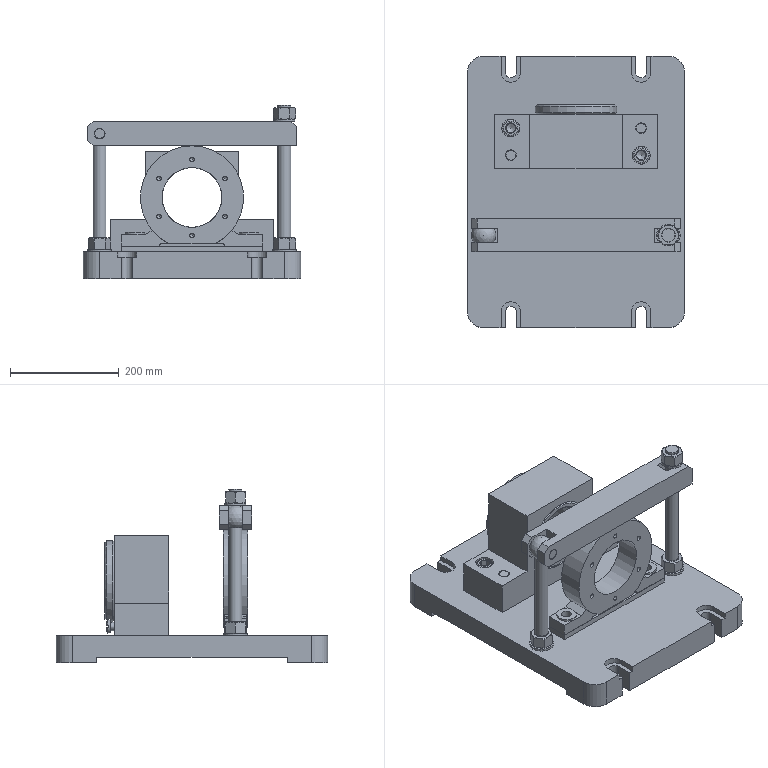Assembly | NX | mm | 21 component files | 21 solids | 393 faces | box 400 x 500 x 320 mm | volume 13709940 mm3 | plane 197 | cylinder 96 | cone 95 | torus 4 | sphere 1 | commonest cylinder face diameters 20 x16 8.5 x12 18 x9 24 x8 21.564 x6 36 x6 10 x4 16 x4
Bill of materials:
unnamed part 1 | 1 |  | Block-style support with a large horizontal cylindrical through-bore in a raised rectangular upright, sitting on a wider rectangular base with flanges extending to both sides.
GB-T848-2002,M24 | 1 |  | Flat annular ring (washer-like disc): a thin cylindrical plate with a single concentric circular through-hole and plain flat faces.
GB-T70.1-2000,M20x70 | 2 |  | Hexagon Socket Head Cap Screw, GB-T 70.1-2000,M20x70
GB-T6170_F-2000,M24x3 | 3 |  | Hexagonal prism with a central round through-hole and chamfered or curved corner faces at both ends; it looks like a hex nut.
GB-T97_1-2002,M24 | 2 |  | Flat annular ring (washer-like disc): a thin cylindrical plate with a single concentric circular through-hole and plain flat faces. Its bore is proportionally smaller than unnamed part's.
unnamed part 2 | 1 |  | Stepped cylindrical pin with a flat round head that has a straight slot, a larger-diameter shoulder below the head, a narrow neck or groove, and a smaller shank with a chamfered end.
unnamed part 3 | 1 |  | Long slender cylindrical rod ending in a rounded, roughly spherical eye with a cross-hole. Near the other end the shaft has a short reduced-diameter section, shown as one or more grooves or steps.
GB-T119.1-2000,20x60 | 1 |  | Parallel Pin, GB-T 119.1-2000,20x60
GB-T119.1-2000,20x90 | 2 |  | Parallel Pin, GB-T 119.1-2000,20x90
unnamed part 4 | 1 |  | Long flat rectangular bar with a slotted fork (clevis-style) at each end. Each fork has a transverse cross-hole, and the end corners are chamfered.
unnamed part 5 | 1 |  | Solid stepped cylindrical pin with a wider central flange or collar, cylindrical sections on both sides, small necks or undercuts next to the collar, and chamfered ends.
unnamed part 6 | 1 |  | Long slender cylindrical pin with chamfered ends and reduced-diameter sections, such as grooves or steps, near both ends.
unnamed part 7 | 1 |  | Stepped cylindrical pin with a central flange or collar. One end has two parallel flats, and the other end is a plain cylinder with a chamfered end.
unnamed part 8 | 1 |  | Housing shaped like a pillow block: a thick annular ring with a large central bore, joined to a two-ear rectangular base. Each ear has a bolt hole with a counterbore or spot face.
unnamed part 9 | 1 |  | Thin-walled cylindrical sleeve with a thin outer flange at one end. Both ends are chamfered.
unnamed part 10 | 1 |  | Rectangular plate with rounded corners. It has four open U-slots on two opposite edges, several through-holes (some countersunk or counterbored), a long raised or recessed strip, and stepped edges on the underside.
Mates:
1. concentric | diamond_pin 1 edge | fixture_body 1 edge
2. concentric | dowel_pin 1 edge | fixture_body 1 edge
3. fix | fixture_body 1 component
4. concentric | bearing_housing 1 edge | fixture_body 1 edge
5. concentric | hinge_screw 1 edge | clamp_plate 1 edge
6. touch align | fix_screw 1 face | fixture_body 1 face
7. touch align | hinge_screw 1 face | fixture_body 1 face
8. touch align | clamp_plate 1 face | bearing_housing 1 face
9. distance | fix_screw 1 face | clamp_plate 1 face
10. concentric | bore_bushing 1 edge | jig_plate 1 edge
11. touch align | bore_bushing 1 face | bearing_housing 1 face
12. distance | jig_plate 1 face | bearing_housing 1 face
13. concentric | bushing_screw 1 edge | jig_plate 1 arc
14. concentric | GB-T848-2002_M24 1 edge | GB-T6170_F-2000_M24x3 1 edge
15. touch align | GB-T848-2002_M24 1 face | fix_screw 1 face
16. touch align | GB-T848-2002_M24 1 face | clamp_plate 1 face
17. concentric | GB-T97_1-2002_M24 2 edge | fixture_body 1 arc
18. concentric | GB-T97_1-2002_M24 1 edge | fixture_body 1 arc
19. concentric | GB-T6170_F-2000_M24x3 3 edge | GB-T97_1-2002_M24 2 edge
20. concentric | GB-T6170_F-2000_M24x3 2 edge | GB-T97_1-2002_M24 1 edge